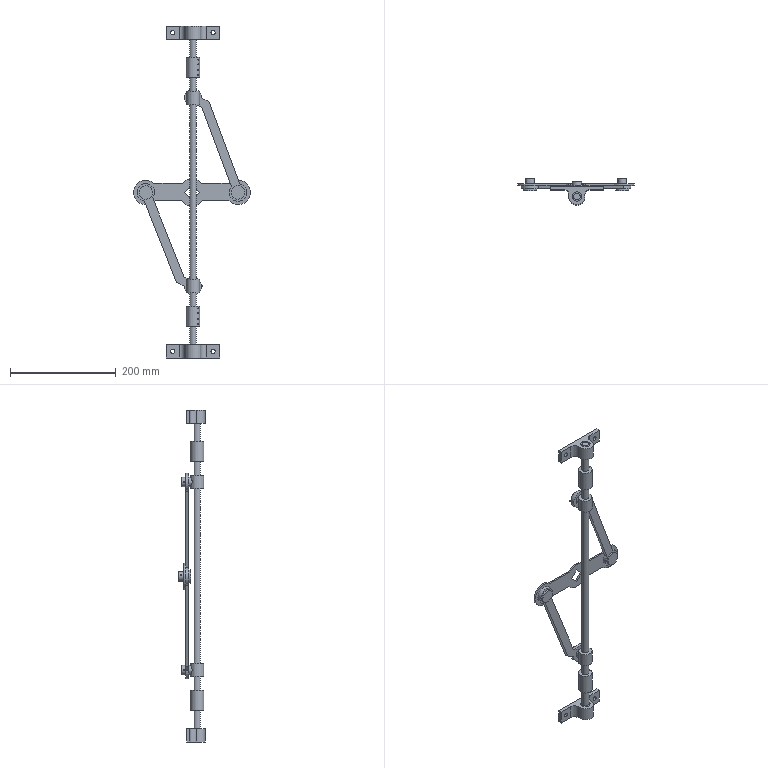Assembly | NX | mm | 24 component files | 24 solids | 391 faces | box 220.84 x 49.44 x 627 mm | volume 289802 mm3 | plane 198 | cylinder 107 | cone 64 | torus 20 | spline 2 | commonest cylinder face diameters 17.78 x14 25.4 x14 2.013 x8 4.5 x8 2.7 x8 5 x8 2.05 x8 12.7 x7
Bill of materials:
unnamed part 1 | 1 |  | Long, slender solid cylindrical rod with plain flat ends.
unnamed part 2 | 2 |  | Tee-shaped body: short thick-walled cylinder with a through bore along its axis, plus a smaller cylindrical arm sticking out sideways at right angles, with a small cross hole near the arm's end.
unnamed part 3 | 2 |  | Headed cylindrical pin: solid cylindrical shank with a larger, thin disc-shaped head at one end and one small hole through the shank near the free end.
unnamed part 4 | 2 |  | Thick-walled cylindrical sleeve with a central bore and one narrow slit along its full length through one side of the wall, making a C-shaped cross-section, plus a row of four evenly spaced holes or pockets along the side next to the slit.
unnamed part 5 | 1 |  | Thin flat plate link with three round lobes joined by straight webs: a round hole in each end lobe and a square hole turned 45 degrees (diamond) in the center lobe.
unnamed part 6 | 2 |  | Plain cylindrical tube or sleeve: a short hollow cylinder with a fairly thin wall and a straight through bore.
unnamed part 7 | 2 |  | Thin flat link of constant thickness with a round eye at each end, each with a hole. The straight web has an offset bend in the plane near one end.
unnamed part 8 | 2 |  | Bracket made as a straight extrusion: a flat rectangular plate with two through holes, joined by fillets to a centered ring-shaped boss with a bore parallel to the plate face.
GB-T70.1-2000,M2.5x10 | 8 |  | Hexagon Socket Head Cap Screw, GB-T 70.1-2000,M2.5x10
GB-T91-2000,2.9x25 | 2 |  | Split Pin, GB-T 91-2000,2.9x25
Mates:
1. concentric | sleeve 2 edge | bracket 2 edge
2. fix | shaft 1 component
3. concentric | bracket 2 edge | shaft 1 edge
4. bond | bracket 2 component | assembly component
5. bond | bracket 2 component | assembly component
6. bond | sleeve 2 component | assembly component
7. bond | bracket 1 component | assembly component
8. bond | sleeve 1 component | assembly component
9. linear | assembly datumaxis | assembly cartesiancoordinatesystem | assembly cartesiancoordinatesystem
10. linear | assembly datumaxis | assembly cartesiancoordinatesystem | assembly cartesiancoordinatesystem
11. concentric | link 2 edge | rod 1 edge
12. concentric | link 1 edge | rod 1 edge
13. concentric | pin_shaft 2 edge | link 2 edge
14. concentric | pin_shaft 1 edge | link 1 edge
15. touch align | shaft_seat 2 face | shaft 1 face
16. touch align | shaft_seat 1 face | shaft 1 face
17. touch align | link 2 face | shaft_seat 2 face
18. touch align | link 1 face | shaft_seat 1 face
19. distance | link 1 face | shaft_seat 1 face
20. center | shaft_seat 2 face | shaft_seat 1 face | bracket 2 face | bracket 1 face
21. parallel | rod 1 face | bracket 1 face
22. touch align | bushing 2 face | shaft 1 face
23. bond | bracket 2 component | assembly component
24. bond | bushing 2 component | assembly component
25. bond | screw_M2_5x10 8 component | assembly component
26. bond | screw_M2_5x10 5 component | assembly component
27. bond | screw_M2_5x10 6 component | assembly component
28. bond | screw_M2_5x10 7 component | assembly component
29. bond | bushing 1 component | assembly component
30. bond | screw_M2_5x10 4 component | assembly component
31. bond | screw_M2_5x10 3 component | assembly component
32. bond | screw_M2_5x10 2 component | assembly component
33. bond | screw_M2_5x10 1 component | assembly component
34. linear | assembly datumaxis | assembly cartesiancoordinatesystem | assembly cartesiancoordinatesystem
35. linear | assembly datumaxis | assembly cartesiancoordinatesystem | assembly cartesiancoordinatesystem
36. linear | assembly datumaxis | assembly cartesiancoordinatesystem | assembly cartesiancoordinatesystem
37. linear | assembly datumaxis | assembly cartesiancoordinatesystem | assembly cartesiancoordinatesystem
38. linear | assembly datumaxis | assembly cartesiancoordinatesystem | assembly cartesiancoordinatesystem